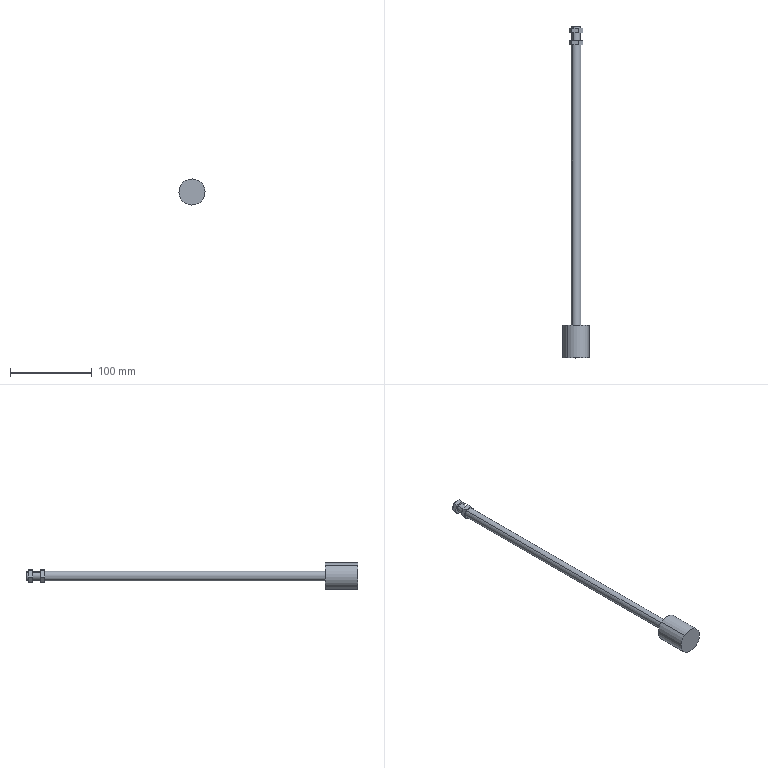Component | SolidWorks | A4-SDA 32X300-KC-L-1_A4-SDA 32X300-KC-L2-1 | 1 solid | 29 faces | box 32 x 407 x 32 mm | volume 73970 mm3 | plane 19 | cylinder 8 | cone 2 | commonest cylinder face diameters 10 x4 12 x2 32 x2
STEP:
#1=COLOUR_RGB('',0.7922,0.8196,0.9333);
#2=FILL_AREA_STYLE_COLOUR('',#1);
#3=FILL_AREA_STYLE('',(#2));
#4=SURFACE_STYLE_FILL_AREA(#3);
#5=SURFACE_SIDE_STYLE('',(#4));
#6=SURFACE_STYLE_USAGE(.BOTH.,#5);
#7=PRESENTATION_STYLE_ASSIGNMENT((#6));
#8=CARTESIAN_POINT('',(-0.1108,13.819,1.359));
#9=VERTEX_POINT('',#8);
#10=CARTESIAN_POINT('',(0.1108,13.819,1.082));
#11=VERTEX_POINT('',#10);
#12=CARTESIAN_POINT('',(-0.,13.819,1.22));
#13=DIRECTION('',(-0.,1.,0.));
#14=DIRECTION('',(-0.6255,0.,0.7802));
#15=AXIS2_PLACEMENT_3D('',#12,#13,#14);
#16=CIRCLE('',#15,0.1772);
#17=EDGE_CURVE('',#9,#11,#16,.T.);
#18=ORIENTED_EDGE('',*,*,#17,.F.);
#19=CARTESIAN_POINT('',(-0.1231,13.799,1.374));
#20=VERTEX_POINT('',#19);
#21=CARTESIAN_POINT('',(-0.1108,13.819,1.359));
#22=DIRECTION('',(-0.4423,-0.7071,0.5517));
#23=VECTOR('',#22,39.37);
#24=LINE('',#21,#23);
#25=EDGE_CURVE('',#9,#20,#24,.T.);
#26=ORIENTED_EDGE('',*,*,#25,.T.);
#27=CARTESIAN_POINT('',(0.1231,13.799,1.067));
#28=VERTEX_POINT('',#27);
#29=CARTESIAN_POINT('',(-0.,13.799,1.22));
#30=DIRECTION('',(0.,-1.,-0.));
#31=DIRECTION('',(-0.6255,0.,0.7802));
#32=AXIS2_PLACEMENT_3D('',#29,#30,#31);
#33=CIRCLE('',#32,0.1969);
#34=EDGE_CURVE('',#28,#20,#33,.T.);
#35=ORIENTED_EDGE('',*,*,#34,.F.);
#36=CARTESIAN_POINT('',(0.1108,13.819,1.082));
#37=DIRECTION('',(0.4423,-0.7071,-0.5517));
#38=VECTOR('',#37,39.37);
#39=LINE('',#36,#38);
#40=EDGE_CURVE('',#11,#28,#39,.T.);
#41=ORIENTED_EDGE('',*,*,#40,.F.);
#42=EDGE_LOOP('',(#18,#26,#35,#41));
#43=FACE_OUTER_BOUND('',#42,.T.);
#44=CARTESIAN_POINT('',(-0.,13.819,1.22));
#45=DIRECTION('',(0.,-1.,-0.));
#46=DIRECTION('',(0.6255,0.,-0.7802));
#47=AXIS2_PLACEMENT_3D('',#44,#45,#46);
#48=CONICAL_SURFACE('',#47,0.1772,0.7854);
#49=ADVANCED_FACE('',(#43),#48,.T.);
#50=CARTESIAN_POINT('',(-0.1478,12.913,1.405));
#51=VERTEX_POINT('',#50);
#52=CARTESIAN_POINT('',(0.1478,12.913,1.036));
#53=VERTEX_POINT('',#52);
#54=CARTESIAN_POINT('',(-0.,12.913,1.22));
#55=DIRECTION('',(-0.,1.,0.));
#56=DIRECTION('',(-0.6255,0.,0.7802));
#57=AXIS2_PLACEMENT_3D('',#54,#55,#56);
#58=CIRCLE('',#57,0.2362);
#59=EDGE_CURVE('',#51,#53,#58,.T.);
#60=ORIENTED_EDGE('',*,*,#59,.F.);
#61=CARTESIAN_POINT('',(-0.1478,-0.6299,1.405));
#62=VERTEX_POINT('',#61);
#63=CARTESIAN_POINT('',(-0.1478,12.913,1.405));
#64=DIRECTION('',(0.,-1.,-0.));
#65=VECTOR('',#64,39.37);
#66=LINE('',#63,#65);
#67=EDGE_CURVE('',#51,#62,#66,.T.);
#68=ORIENTED_EDGE('',*,*,#67,.T.);
#69=CARTESIAN_POINT('',(0.1478,-0.6299,1.036));
#70=VERTEX_POINT('',#69);
#71=CARTESIAN_POINT('',(0.,-0.6299,1.22));
#72=DIRECTION('',(-0.,1.,0.));
#73=DIRECTION('',(-0.6255,0.,0.7802));
#74=AXIS2_PLACEMENT_3D('',#71,#72,#73);
#75=CIRCLE('',#74,0.2362);
#76=EDGE_CURVE('',#62,#70,#75,.T.);
#77=ORIENTED_EDGE('',*,*,#76,.T.);
#78=CARTESIAN_POINT('',(0.1478,12.913,1.036));
#79=DIRECTION('',(0.,-1.,-0.));
#80=VECTOR('',#79,39.37);
#81=LINE('',#78,#80);
#82=EDGE_CURVE('',#53,#70,#81,.T.);
#83=ORIENTED_EDGE('',*,*,#82,.F.);
#84=EDGE_LOOP('',(#60,#68,#77,#83));
#85=FACE_OUTER_BOUND('',#84,.T.);
#86=CARTESIAN_POINT('',(-0.,12.913,1.22));
#87=DIRECTION('',(0.,-1.,-0.));
#88=DIRECTION('',(0.6255,0.,-0.7802));
#89=AXIS2_PLACEMENT_3D('',#86,#87,#88);
#90=CYLINDRICAL_SURFACE('',#89,0.2362);
#91=ADVANCED_FACE('',(#85),#90,.T.);
#92=CARTESIAN_POINT('',(-0.394,-2.205,1.712));
#93=VERTEX_POINT('',#92);
#94=CARTESIAN_POINT('',(0.394,-2.205,0.729));
#95=VERTEX_POINT('',#94);
#96=CARTESIAN_POINT('',(0.,-2.205,1.22));
#97=DIRECTION('',(-0.,1.,0.));
#98=DIRECTION('',(-0.6255,-0.,0.7802));
#99=AXIS2_PLACEMENT_3D('',#96,#97,#98);
#100=CIRCLE('',#99,0.6299);
#101=EDGE_CURVE('',#93,#95,#100,.T.);
#102=ORIENTED_EDGE('',*,*,#101,.T.);
#103=CARTESIAN_POINT('',(0.394,-0.6299,0.729));
#104=VERTEX_POINT('',#103);
#105=CARTESIAN_POINT('',(0.394,-2.205,0.729));
#106=DIRECTION('',(-0.,1.,0.));
#107=VECTOR('',#106,39.37);
#108=LINE('',#105,#107);
#109=EDGE_CURVE('',#95,#104,#108,.T.);
#110=ORIENTED_EDGE('',*,*,#109,.T.);
#111=CARTESIAN_POINT('',(-0.394,-0.6299,1.712));
#112=VERTEX_POINT('',#111);
#113=CARTESIAN_POINT('',(0.,-0.6299,1.22));
#114=DIRECTION('',(-0.,1.,0.));
#115=DIRECTION('',(-0.6255,-0.,0.7802));
#116=AXIS2_PLACEMENT_3D('',#113,#114,#115);
#117=CIRCLE('',#116,0.6299);
#118=EDGE_CURVE('',#112,#104,#117,.T.);
#119=ORIENTED_EDGE('',*,*,#118,.F.);
#120=CARTESIAN_POINT('',(-0.394,-2.205,1.712));
#121=DIRECTION('',(-0.,1.,0.));
#122=VECTOR('',#121,39.37);
#123=LINE('',#120,#122);
#124=EDGE_CURVE('',#93,#112,#123,.T.);
#125=ORIENTED_EDGE('',*,*,#124,.F.);
#126=EDGE_LOOP('',(#102,#110,#119,#125));
#127=FACE_OUTER_BOUND('',#126,.T.);
#128=CARTESIAN_POINT('',(0.,-2.205,1.22));
#129=DIRECTION('',(-0.,1.,0.));
#130=DIRECTION('',(-0.6255,-0.,0.7802));
#131=AXIS2_PLACEMENT_3D('',#128,#129,#130);
#132=CYLINDRICAL_SURFACE('',#131,0.6299);
#133=ADVANCED_FACE('',(#127),#132,.T.);
#134=ORIENTED_EDGE('',*,*,#34,.T.);
#135=CARTESIAN_POINT('',(-0.1231,13.701,1.374));
#136=VERTEX_POINT('',#135);
#137=CARTESIAN_POINT('',(-0.1231,13.819,1.374));
#138=DIRECTION('',(0.,-1.,-0.));
#139=VECTOR('',#138,39.37);
#140=LINE('',#137,#139);
#141=EDGE_CURVE('',#20,#136,#140,.T.);
#142=ORIENTED_EDGE('',*,*,#141,.T.);
#143=CARTESIAN_POINT('',(0.1231,13.701,1.067));
#144=VERTEX_POINT('',#143);
#145=CARTESIAN_POINT('',(-0.,13.701,1.22));
#146=DIRECTION('',(0.,-1.,-0.));
#147=DIRECTION('',(0.6255,0.,-0.7802));
#148=AXIS2_PLACEMENT_3D('',#145,#146,#147);
#149=CIRCLE('',#148,0.1969);
#150=EDGE_CURVE('',#144,#136,#149,.T.);
#151=ORIENTED_EDGE('',*,*,#150,.F.);
#152=CARTESIAN_POINT('',(0.1231,13.819,1.067));
#153=DIRECTION('',(0.,-1.,-0.));
#154=VECTOR('',#153,39.37);
#155=LINE('',#152,#154);
#156=EDGE_CURVE('',#28,#144,#155,.T.);
#157=ORIENTED_EDGE('',*,*,#156,.F.);
#158=EDGE_LOOP('',(#134,#142,#151,#157));
#159=FACE_OUTER_BOUND('',#158,.T.);
#160=CARTESIAN_POINT('',(-0.,13.819,1.22));
#161=DIRECTION('',(0.,-1.,-0.));
#162=DIRECTION('',(0.6255,0.,-0.7802));
#163=AXIS2_PLACEMENT_3D('',#160,#161,#162);
#164=CYLINDRICAL_SURFACE('',#163,0.1969);
#165=ADVANCED_FACE('',(#159),#164,.T.);
#166=CARTESIAN_POINT('',(0.1231,13.504,1.067));
#167=VERTEX_POINT('',#166);
#168=CARTESIAN_POINT('',(-0.1231,13.504,1.374));
#169=VERTEX_POINT('',#168);
#170=CARTESIAN_POINT('',(-0.,13.504,1.22));
#171=DIRECTION('',(0.,-1.,-0.));
#172=DIRECTION('',(0.6255,0.,-0.7802));
#173=AXIS2_PLACEMENT_3D('',#170,#171,#172);
#174=CIRCLE('',#173,0.1969);
#175=EDGE_CURVE('',#167,#169,#174,.T.);
#176=ORIENTED_EDGE('',*,*,#175,.T.);
#177=CARTESIAN_POINT('',(-0.1231,13.11,1.374));
#178=VERTEX_POINT('',#177);
#179=CARTESIAN_POINT('',(-0.1231,13.819,1.374));
#180=DIRECTION('',(0.,-1.,-0.));
#181=VECTOR('',#180,39.37);
#182=LINE('',#179,#181);
#183=EDGE_CURVE('',#169,#178,#182,.T.);
#184=ORIENTED_EDGE('',*,*,#183,.T.);
#185=CARTESIAN_POINT('',(0.1231,13.11,1.067));
#186=VERTEX_POINT('',#185);
#187=CARTESIAN_POINT('',(-0.,13.11,1.22));
#188=DIRECTION('',(0.,-1.,-0.));
#189=DIRECTION('',(0.6255,0.,-0.7802));
#190=AXIS2_PLACEMENT_3D('',#187,#188,#189);
#191=CIRCLE('',#190,0.1969);
#192=EDGE_CURVE('',#186,#178,#191,.T.);
#193=ORIENTED_EDGE('',*,*,#192,.F.);
#194=CARTESIAN_POINT('',(0.1231,13.819,1.067));
#195=DIRECTION('',(0.,-1.,-0.));
#196=VECTOR('',#195,39.37);
#197=LINE('',#194,#196);
#198=EDGE_CURVE('',#167,#186,#197,.T.);
#199=ORIENTED_EDGE('',*,*,#198,.F.);
#200=EDGE_LOOP('',(#176,#184,#193,#199));
#201=FACE_OUTER_BOUND('',#200,.T.);
#202=CARTESIAN_POINT('',(-0.,13.819,1.22));
#203=DIRECTION('',(0.,-1.,-0.));
#204=DIRECTION('',(0.6255,0.,-0.7802));
#205=AXIS2_PLACEMENT_3D('',#202,#203,#204);
#206=CYLINDRICAL_SURFACE('',#205,0.1969);
#207=ADVANCED_FACE('',(#201),#206,.T.);
#208=ORIENTED_EDGE('',*,*,#183,.F.);
#209=CARTESIAN_POINT('',(-0.,13.504,1.22));
#210=DIRECTION('',(0.,-1.,-0.));
#211=DIRECTION('',(0.6255,0.,-0.7802));
#212=AXIS2_PLACEMENT_3D('',#209,#210,#211);
#213=CIRCLE('',#212,0.1969);
#214=EDGE_CURVE('',#169,#167,#213,.T.);
#215=ORIENTED_EDGE('',*,*,#214,.T.);
#216=ORIENTED_EDGE('',*,*,#198,.T.);
#217=CARTESIAN_POINT('',(-0.,13.11,1.22));
#218=DIRECTION('',(0.,-1.,-0.));
#219=DIRECTION('',(0.6255,0.,-0.7802));
#220=AXIS2_PLACEMENT_3D('',#217,#218,#219);
#221=CIRCLE('',#220,0.1969);
#222=EDGE_CURVE('',#178,#186,#221,.T.);
#223=ORIENTED_EDGE('',*,*,#222,.F.);
#224=EDGE_LOOP('',(#208,#215,#216,#223));
#225=FACE_OUTER_BOUND('',#224,.T.);
#226=CARTESIAN_POINT('',(-0.,13.819,1.22));
#227=DIRECTION('',(0.,-1.,-0.));
#228=DIRECTION('',(0.6255,0.,-0.7802));
#229=AXIS2_PLACEMENT_3D('',#226,#227,#228);
#230=CYLINDRICAL_SURFACE('',#229,0.1969);
#231=ADVANCED_FACE('',(#225),#230,.T.);
#232=CARTESIAN_POINT('',(0.3308,13.504,1.271));
#233=VERTEX_POINT('',#232);
#234=CARTESIAN_POINT('',(0.2093,13.504,0.9594));
#235=VERTEX_POINT('',#234);
#236=CARTESIAN_POINT('',(0.2093,13.504,0.9594));
#237=DIRECTION('',(-0.363,0.,-0.9318));
#238=VECTOR('',#237,39.37);
#239=LINE('',#236,#238);
#240=EDGE_CURVE('',#233,#235,#239,.T.);
#241=ORIENTED_EDGE('',*,*,#240,.F.);
#242=CARTESIAN_POINT('',(0.1215,13.504,1.532));
#243=VERTEX_POINT('',#242);
#244=CARTESIAN_POINT('',(0.3308,13.504,1.271));
#245=DIRECTION('',(0.6255,0.,-0.7802));
#246=VECTOR('',#245,39.37);
#247=LINE('',#244,#246);
#248=EDGE_CURVE('',#243,#233,#247,.T.);
#249=ORIENTED_EDGE('',*,*,#248,.F.);
#250=CARTESIAN_POINT('',(-0.2093,13.504,1.482));
#251=VERTEX_POINT('',#250);
#252=CARTESIAN_POINT('',(0.1215,13.504,1.532));
#253=DIRECTION('',(0.9884,0.,0.1516));
#254=VECTOR('',#253,39.37);
#255=LINE('',#252,#254);
#256=EDGE_CURVE('',#251,#243,#255,.T.);
#257=ORIENTED_EDGE('',*,*,#256,.F.);
#258=CARTESIAN_POINT('',(-0.3308,13.504,1.17));
#259=VERTEX_POINT('',#258);
#260=CARTESIAN_POINT('',(-0.2093,13.504,1.482));
#261=DIRECTION('',(0.363,-0.,0.9318));
#262=VECTOR('',#261,39.37);
#263=LINE('',#260,#262);
#264=EDGE_CURVE('',#259,#251,#263,.T.);
#265=ORIENTED_EDGE('',*,*,#264,.F.);
#266=CARTESIAN_POINT('',(-0.1215,13.504,0.9086));
#267=VERTEX_POINT('',#266);
#268=CARTESIAN_POINT('',(-0.3308,13.504,1.17));
#269=DIRECTION('',(-0.6255,-0.,0.7802));
#270=VECTOR('',#269,39.37);
#271=LINE('',#268,#270);
#272=EDGE_CURVE('',#267,#259,#271,.T.);
#273=ORIENTED_EDGE('',*,*,#272,.F.);
#274=CARTESIAN_POINT('',(-0.1215,13.504,0.9086));
#275=DIRECTION('',(-0.9884,-0.,-0.1516));
#276=VECTOR('',#275,39.37);
#277=LINE('',#274,#276);
#278=EDGE_CURVE('',#235,#267,#277,.T.);
#279=ORIENTED_EDGE('',*,*,#278,.F.);
#280=EDGE_LOOP('',(#241,#249,#257,#265,#273,#279));
#281=FACE_OUTER_BOUND('',#280,.T.);
#282=ORIENTED_EDGE('',*,*,#175,.F.);
#283=ORIENTED_EDGE('',*,*,#214,.F.);
#284=EDGE_LOOP('',(#282,#283));
#285=FACE_BOUND('',#284,.T.);
#286=CARTESIAN_POINT('',(-0.,13.504,1.22));
#287=DIRECTION('',(0.,-1.,-0.));
#288=DIRECTION('',(0.6255,0.,-0.7802));
#289=AXIS2_PLACEMENT_3D('',#286,#287,#288);
#290=PLANE('',#289);
#291=ADVANCED_FACE('',(#281,#285),#290,.T.);
#292=CARTESIAN_POINT('',(0.3308,13.701,1.271));
#293=VERTEX_POINT('',#292);
#294=CARTESIAN_POINT('',(0.2093,13.701,0.9594));
#295=VERTEX_POINT('',#294);
#296=CARTESIAN_POINT('',(0.2093,13.701,0.9594));
#297=DIRECTION('',(-0.363,0.,-0.9318));
#298=VECTOR('',#297,39.37);
#299=LINE('',#296,#298);
#300=EDGE_CURVE('',#293,#295,#299,.T.);
#301=ORIENTED_EDGE('',*,*,#300,.T.);
#302=CARTESIAN_POINT('',(-0.1215,13.701,0.9086));
#303=VERTEX_POINT('',#302);
#304=CARTESIAN_POINT('',(-0.1215,13.701,0.9086));
#305=DIRECTION('',(-0.9884,-0.,-0.1516));
#306=VECTOR('',#305,39.37);
#307=LINE('',#304,#306);
#308=EDGE_CURVE('',#295,#303,#307,.T.);
#309=ORIENTED_EDGE('',*,*,#308,.T.);
#310=CARTESIAN_POINT('',(-0.3308,13.701,1.17));
#311=VERTEX_POINT('',#310);
#312=CARTESIAN_POINT('',(-0.3308,13.701,1.17));
#313=DIRECTION('',(-0.6255,-0.,0.7802));
#314=VECTOR('',#313,39.37);
#315=LINE('',#312,#314);
#316=EDGE_CURVE('',#303,#311,#315,.T.);
#317=ORIENTED_EDGE('',*,*,#316,.T.);
#318=CARTESIAN_POINT('',(-0.2093,13.701,1.482));
#319=VERTEX_POINT('',#318);
#320=CARTESIAN_POINT('',(-0.2093,13.701,1.482));
#321=DIRECTION('',(0.363,-0.,0.9318));
#322=VECTOR('',#321,39.37);
#323=LINE('',#320,#322);
#324=EDGE_CURVE('',#311,#319,#323,.T.);
#325=ORIENTED_EDGE('',*,*,#324,.T.);
#326=CARTESIAN_POINT('',(0.1215,13.701,1.532));
#327=VERTEX_POINT('',#326);
#328=CARTESIAN_POINT('',(0.1215,13.701,1.532));
#329=DIRECTION('',(0.9884,0.,0.1516));
#330=VECTOR('',#329,39.37);
#331=LINE('',#328,#330);
#332=EDGE_CURVE('',#319,#327,#331,.T.);
#333=ORIENTED_EDGE('',*,*,#332,.T.);
#334=CARTESIAN_POINT('',(0.3308,13.701,1.271));
#335=DIRECTION('',(0.6255,0.,-0.7802));
#336=VECTOR('',#335,39.37);
#337=LINE('',#334,#336);
#338=EDGE_CURVE('',#327,#293,#337,.T.);
#339=ORIENTED_EDGE('',*,*,#338,.T.);
#340=EDGE_LOOP('',(#301,#309,#317,#325,#333,#339));
#341=FACE_OUTER_BOUND('',#340,.T.);
#342=ORIENTED_EDGE('',*,*,#150,.T.);
#343=CARTESIAN_POINT('',(-0.,13.701,1.22));
#344=DIRECTION('',(0.,-1.,-0.));
#345=DIRECTION('',(0.6255,0.,-0.7802));
#346=AXIS2_PLACEMENT_3D('',#343,#344,#345);
#347=CIRCLE('',#346,0.1969);
#348=EDGE_CURVE('',#136,#144,#347,.T.);
#349=ORIENTED_EDGE('',*,*,#348,.T.);
#350=EDGE_LOOP('',(#342,#349));
#351=FACE_BOUND('',#350,.T.);
#352=CARTESIAN_POINT('',(-0.,13.701,1.22));
#353=DIRECTION('',(0.,-1.,-0.));
#354=DIRECTION('',(0.6255,0.,-0.7802));
#355=AXIS2_PLACEMENT_3D('',#352,#353,#354);
#356=PLANE('',#355);
#357=ADVANCED_FACE('',(#341,#351),#356,.F.);
#358=ORIENTED_EDGE('',*,*,#300,.F.);
#359=CARTESIAN_POINT('',(0.3308,13.504,1.271));
#360=DIRECTION('',(-0.,1.,0.));
#361=VECTOR('',#360,39.37);
#362=LINE('',#359,#361);
#363=EDGE_CURVE('',#233,#293,#362,.T.);
#364=ORIENTED_EDGE('',*,*,#363,.F.);
#365=ORIENTED_EDGE('',*,*,#240,.T.);
#366=CARTESIAN_POINT('',(0.2093,13.504,0.9594));
#367=DIRECTION('',(-0.,1.,0.));
#368=VECTOR('',#367,39.37);
#369=LINE('',#366,#368);
#370=EDGE_CURVE('',#235,#295,#369,.T.);
#371=ORIENTED_EDGE('',*,*,#370,.T.);
#372=EDGE_LOOP('',(#358,#364,#365,#371));
#373=FACE_OUTER_BOUND('',#372,.T.);
#374=CARTESIAN_POINT('',(0.2093,13.504,0.9594));
#375=DIRECTION('',(0.9318,0.,-0.363));
#376=DIRECTION('',(-0.363,0.,-0.9318));
#377=AXIS2_PLACEMENT_3D('',#374,#375,#376);
#378=PLANE('',#377);
#379=ADVANCED_FACE('',(#373),#378,.T.);
#380=ORIENTED_EDGE('',*,*,#338,.F.);
#381=CARTESIAN_POINT('',(0.1215,13.504,1.532));
#382=DIRECTION('',(-0.,1.,0.));
#383=VECTOR('',#382,39.37);
#384=LINE('',#381,#383);
#385=EDGE_CURVE('',#243,#327,#384,.T.);
#386=ORIENTED_EDGE('',*,*,#385,.F.);
#387=ORIENTED_EDGE('',*,*,#248,.T.);
#388=ORIENTED_EDGE('',*,*,#363,.T.);
#389=EDGE_LOOP('',(#380,#386,#387,#388));
#390=FACE_OUTER_BOUND('',#389,.T.);
#391=CARTESIAN_POINT('',(0.3308,13.504,1.271));
#392=DIRECTION('',(0.7802,0.,0.6255));
#393=DIRECTION('',(-0.,1.,0.));
#394=AXIS2_PLACEMENT_3D('',#391,#392,#393);
#395=PLANE('',#394);
#396=ADVANCED_FACE('',(#390),#395,.T.);
#397=ORIENTED_EDGE('',*,*,#332,.F.);
#398=CARTESIAN_POINT('',(-0.2093,13.504,1.482));
#399=DIRECTION('',(-0.,1.,0.));
#400=VECTOR('',#399,39.37);
#401=LINE('',#398,#400);
#402=EDGE_CURVE('',#251,#319,#401,.T.);
#403=ORIENTED_EDGE('',*,*,#402,.F.);
#404=ORIENTED_EDGE('',*,*,#256,.T.);
#405=ORIENTED_EDGE('',*,*,#385,.T.);
#406=EDGE_LOOP('',(#397,#403,#404,#405));
#407=FACE_OUTER_BOUND('',#406,.T.);
#408=CARTESIAN_POINT('',(0.1215,13.504,1.532));
#409=DIRECTION('',(-0.1516,-0.,0.9884));
#410=DIRECTION('',(0.9884,0.,0.1516));
#411=AXIS2_PLACEMENT_3D('',#408,#409,#410);
#412=PLANE('',#411);
#413=ADVANCED_FACE('',(#407),#412,.T.);
#414=ORIENTED_EDGE('',*,*,#324,.F.);
#415=CARTESIAN_POINT('',(-0.3308,13.504,1.17));
#416=DIRECTION('',(-0.,1.,0.));
#417=VECTOR('',#416,39.37);
#418=LINE('',#415,#417);
#419=EDGE_CURVE('',#259,#311,#418,.T.);
#420=ORIENTED_EDGE('',*,*,#419,.F.);
#421=ORIENTED_EDGE('',*,*,#264,.T.);
#422=ORIENTED_EDGE('',*,*,#402,.T.);
#423=EDGE_LOOP('',(#414,#420,#421,#422));
#424=FACE_OUTER_BOUND('',#423,.T.);
#425=CARTESIAN_POINT('',(-0.2093,13.504,1.482));
#426=DIRECTION('',(-0.9318,-0.,0.363));
#427=DIRECTION('',(0.363,-0.,0.9318));
#428=AXIS2_PLACEMENT_3D('',#425,#426,#427);
#429=PLANE('',#428);
#430=ADVANCED_FACE('',(#424),#429,.T.);
#431=ORIENTED_EDGE('',*,*,#316,.F.);
#432=CARTESIAN_POINT('',(-0.1215,13.504,0.9086));
#433=DIRECTION('',(-0.,1.,0.));
#434=VECTOR('',#433,39.37);
#435=LINE('',#432,#434);
#436=EDGE_CURVE('',#267,#303,#435,.T.);
#437=ORIENTED_EDGE('',*,*,#436,.F.);
#438=ORIENTED_EDGE('',*,*,#272,.T.);
#439=ORIENTED_EDGE('',*,*,#419,.T.);
#440=EDGE_LOOP('',(#431,#437,#438,#439));
#441=FACE_OUTER_BOUND('',#440,.T.);
#442=CARTESIAN_POINT('',(-0.3308,13.504,1.17));
#443=DIRECTION('',(-0.7802,-0.,-0.6255));
#444=DIRECTION('',(0.,-1.,-0.));
#445=AXIS2_PLACEMENT_3D('',#442,#443,#444);
#446=PLANE('',#445);
#447=ADVANCED_FACE('',(#441),#446,.T.);
#448=ORIENTED_EDGE('',*,*,#308,.F.);
#449=ORIENTED_EDGE('',*,*,#370,.F.);
#450=ORIENTED_EDGE('',*,*,#278,.T.);
#451=ORIENTED_EDGE('',*,*,#436,.T.);
#452=EDGE_LOOP('',(#448,#449,#450,#451));
#453=FACE_OUTER_BOUND('',#452,.T.);
#454=CARTESIAN_POINT('',(-0.1215,13.504,0.9086));
#455=DIRECTION('',(0.1516,0.,-0.9884));
#456=DIRECTION('',(-0.9884,-0.,-0.1516));
#457=AXIS2_PLACEMENT_3D('',#454,#455,#456);
#458=PLANE('',#457);
#459=ADVANCED_FACE('',(#453),#458,.T.);
#460=CARTESIAN_POINT('',(-0.,13.819,1.22));
#461=DIRECTION('',(-0.,1.,0.));
#462=DIRECTION('',(-0.6255,0.,0.7802));
#463=AXIS2_PLACEMENT_3D('',#460,#461,#462);
#464=CIRCLE('',#463,0.1772);
#465=EDGE_CURVE('',#11,#9,#464,.T.);
#466=ORIENTED_EDGE('',*,*,#465,.T.);
#467=ORIENTED_EDGE('',*,*,#17,.T.);
#468=EDGE_LOOP('',(#466,#467));
#469=FACE_OUTER_BOUND('',#468,.T.);
#470=CARTESIAN_POINT('',(-0.,13.819,1.22));
#471=DIRECTION('',(-0.,1.,0.));
#472=DIRECTION('',(-0.6255,-0.,0.7802));
#473=AXIS2_PLACEMENT_3D('',#470,#471,#472);
#474=PLANE('',#473);
#475=ADVANCED_FACE('',(#469),#474,.T.);
#476=ORIENTED_EDGE('',*,*,#141,.F.);
#477=CARTESIAN_POINT('',(-0.,13.799,1.22));
#478=DIRECTION('',(0.,-1.,-0.));
#479=DIRECTION('',(-0.6255,0.,0.7802));
#480=AXIS2_PLACEMENT_3D('',#477,#478,#479);
#481=CIRCLE('',#480,0.1969);
#482=EDGE_CURVE('',#20,#28,#481,.T.);
#483=ORIENTED_EDGE('',*,*,#482,.T.);
#484=ORIENTED_EDGE('',*,*,#156,.T.);
#485=ORIENTED_EDGE('',*,*,#348,.F.);
#486=EDGE_LOOP('',(#476,#483,#484,#485));
#487=FACE_OUTER_BOUND('',#486,.T.);
#488=CARTESIAN_POINT('',(-0.,13.819,1.22));
#489=DIRECTION('',(0.,-1.,-0.));
#490=DIRECTION('',(0.6255,0.,-0.7802));
#491=AXIS2_PLACEMENT_3D('',#488,#489,#490);
#492=CYLINDRICAL_SURFACE('',#491,0.1969);
#493=ADVANCED_FACE('',(#487),#492,.T.);
#494=CARTESIAN_POINT('',(0.3308,12.913,1.271));
#495=VERTEX_POINT('',#494);
#496=CARTESIAN_POINT('',(0.2093,12.913,0.9594));
#497=VERTEX_POINT('',#496);
#498=CARTESIAN_POINT('',(0.2093,12.913,0.9594));
#499=DIRECTION('',(-0.363,0.,-0.9318));
#500=VECTOR('',#499,39.37);
#501=LINE('',#498,#500);
#502=EDGE_CURVE('',#495,#497,#501,.T.);
#503=ORIENTED_EDGE('',*,*,#502,.F.);
#504=CARTESIAN_POINT('',(0.1215,12.913,1.532));
#505=VERTEX_POINT('',#504);
#506=CARTESIAN_POINT('',(0.3308,12.913,1.271));
#507=DIRECTION('',(0.6255,0.,-0.7802));
#508=VECTOR('',#507,39.37);
#509=LINE('',#506,#508);
#510=EDGE_CURVE('',#505,#495,#509,.T.);
#511=ORIENTED_EDGE('',*,*,#510,.F.);
#512=CARTESIAN_POINT('',(-0.2093,12.913,1.482));
#513=VERTEX_POINT('',#512);
#514=CARTESIAN_POINT('',(0.1215,12.913,1.532));
#515=DIRECTION('',(0.9884,0.,0.1516));
#516=VECTOR('',#515,39.37);
#517=LINE('',#514,#516);
#518=EDGE_CURVE('',#513,#505,#517,.T.);
#519=ORIENTED_EDGE('',*,*,#518,.F.);
#520=CARTESIAN_POINT('',(-0.3308,12.913,1.17));
#521=VERTEX_POINT('',#520);
#522=CARTESIAN_POINT('',(-0.2093,12.913,1.482));
#523=DIRECTION('',(0.363,-0.,0.9318));
#524=VECTOR('',#523,39.37);
#525=LINE('',#522,#524);
#526=EDGE_CURVE('',#521,#513,#525,.T.);
#527=ORIENTED_EDGE('',*,*,#526,.F.);
#528=CARTESIAN_POINT('',(-0.1215,12.913,0.9086));
#529=VERTEX_POINT('',#528);
#530=CARTESIAN_POINT('',(-0.3308,12.913,1.17));
#531=DIRECTION('',(-0.6255,-0.,0.7802));
#532=VECTOR('',#531,39.37);
#533=LINE('',#530,#532);
#534=EDGE_CURVE('',#529,#521,#533,.T.);
#535=ORIENTED_EDGE('',*,*,#534,.F.);
#536=CARTESIAN_POINT('',(-0.1215,12.913,0.9086));
#537=DIRECTION('',(-0.9884,-0.,-0.1516));
#538=VECTOR('',#537,39.37);
#539=LINE('',#536,#538);
#540=EDGE_CURVE('',#497,#529,#539,.T.);
#541=ORIENTED_EDGE('',*,*,#540,.F.);
#542=EDGE_LOOP('',(#503,#511,#519,#527,#535,#541));
#543=FACE_OUTER_BOUND('',#542,.T.);
#544=CARTESIAN_POINT('',(-0.,12.913,1.22));
#545=DIRECTION('',(-0.,1.,0.));
#546=DIRECTION('',(-0.6255,0.,0.7802));
#547=AXIS2_PLACEMENT_3D('',#544,#545,#546);
#548=CIRCLE('',#547,0.2362);
#549=EDGE_CURVE('',#53,#51,#548,.T.);
#550=ORIENTED_EDGE('',*,*,#549,.T.);
#551=ORIENTED_EDGE('',*,*,#59,.T.);
#552=EDGE_LOOP('',(#550,#551));
#553=FACE_BOUND('',#552,.T.);
#554=CARTESIAN_POINT('',(-0.,12.913,1.22));
#555=DIRECTION('',(0.,-1.,-0.));
#556=DIRECTION('',(0.6255,0.,-0.7802));
#557=AXIS2_PLACEMENT_3D('',#554,#555,#556);
#558=PLANE('',#557);
#559=ADVANCED_FACE('',(#543,#553),#558,.T.);
#560=CARTESIAN_POINT('',(0.3308,13.11,1.271));
#561=VERTEX_POINT('',#560);
#562=CARTESIAN_POINT('',(0.2093,13.11,0.9594));
#563=VERTEX_POINT('',#562);
#564=CARTESIAN_POINT('',(0.2093,13.11,0.9594));
#565=DIRECTION('',(-0.363,0.,-0.9318));
#566=VECTOR('',#565,39.37);
#567=LINE('',#564,#566);
#568=EDGE_CURVE('',#561,#563,#567,.T.);
#569=ORIENTED_EDGE('',*,*,#568,.T.);
#570=CARTESIAN_POINT('',(-0.1215,13.11,0.9086));
#571=VERTEX_POINT('',#570);
#572=CARTESIAN_POINT('',(-0.1215,13.11,0.9086));
#573=DIRECTION('',(-0.9884,-0.,-0.1516));
#574=VECTOR('',#573,39.37);
#575=LINE('',#572,#574);
#576=EDGE_CURVE('',#563,#571,#575,.T.);
#577=ORIENTED_EDGE('',*,*,#576,.T.);
#578=CARTESIAN_POINT('',(-0.3308,13.11,1.17));
#579=VERTEX_POINT('',#578);
#580=CARTESIAN_POINT('',(-0.3308,13.11,1.17));
#581=DIRECTION('',(-0.6255,-0.,0.7802));
#582=VECTOR('',#581,39.37);
#583=LINE('',#580,#582);
#584=EDGE_CURVE('',#571,#579,#583,.T.);
#585=ORIENTED_EDGE('',*,*,#584,.T.);
#586=CARTESIAN_POINT('',(-0.2093,13.11,1.482));
#587=VERTEX_POINT('',#586);
#588=CARTESIAN_POINT('',(-0.2093,13.11,1.482));
#589=DIRECTION('',(0.363,-0.,0.9318));
#590=VECTOR('',#589,39.37);
#591=LINE('',#588,#590);
#592=EDGE_CURVE('',#579,#587,#591,.T.);
#593=ORIENTED_EDGE('',*,*,#592,.T.);
#594=CARTESIAN_POINT('',(0.1215,13.11,1.532));
#595=VERTEX_POINT('',#594);
#596=CARTESIAN_POINT('',(0.1215,13.11,1.532));
#597=DIRECTION('',(0.9884,0.,0.1516));
#598=VECTOR('',#597,39.37);
#599=LINE('',#596,#598);
#600=EDGE_CURVE('',#587,#595,#599,.T.);
#601=ORIENTED_EDGE('',*,*,#600,.T.);
#602=CARTESIAN_POINT('',(0.3308,13.11,1.271));
#603=DIRECTION('',(0.6255,0.,-0.7802));
#604=VECTOR('',#603,39.37);
#605=LINE('',#602,#604);
#606=EDGE_CURVE('',#595,#561,#605,.T.);
#607=ORIENTED_EDGE('',*,*,#606,.T.);
#608=EDGE_LOOP('',(#569,#577,#585,#593,#601,#607));
#609=FACE_OUTER_BOUND('',#608,.T.);
#610=ORIENTED_EDGE('',*,*,#192,.T.);
#611=ORIENTED_EDGE('',*,*,#222,.T.);
#612=EDGE_LOOP('',(#610,#611));
#613=FACE_BOUND('',#612,.T.);
#614=CARTESIAN_POINT('',(-0.,13.11,1.22));
#615=DIRECTION('',(0.,-1.,-0.));
#616=DIRECTION('',(0.6255,0.,-0.7802));
#617=AXIS2_PLACEMENT_3D('',#614,#615,#616);
#618=PLANE('',#617);
#619=ADVANCED_FACE('',(#609,#613),#618,.F.);
#620=ORIENTED_EDGE('',*,*,#568,.F.);
#621=CARTESIAN_POINT('',(0.3308,12.913,1.271));
#622=DIRECTION('',(-0.,1.,0.));
#623=VECTOR('',#622,39.37);
#624=LINE('',#621,#623);
#625=EDGE_CURVE('',#495,#561,#624,.T.);
#626=ORIENTED_EDGE('',*,*,#625,.F.);
#627=ORIENTED_EDGE('',*,*,#502,.T.);
#628=CARTESIAN_POINT('',(0.2093,12.913,0.9594));
#629=DIRECTION('',(-0.,1.,0.));
#630=VECTOR('',#629,39.37);
#631=LINE('',#628,#630);
#632=EDGE_CURVE('',#497,#563,#631,.T.);
#633=ORIENTED_EDGE('',*,*,#632,.T.);
#634=EDGE_LOOP('',(#620,#626,#627,#633));
#635=FACE_OUTER_BOUND('',#634,.T.);
#636=CARTESIAN_POINT('',(0.2093,12.913,0.9594));
#637=DIRECTION('',(0.9318,0.,-0.363));
#638=DIRECTION('',(-0.363,0.,-0.9318));
#639=AXIS2_PLACEMENT_3D('',#636,#637,#638);
#640=PLANE('',#639);
#641=ADVANCED_FACE('',(#635),#640,.T.);
#642=ORIENTED_EDGE('',*,*,#606,.F.);
#643=CARTESIAN_POINT('',(0.1215,12.913,1.532));
#644=DIRECTION('',(-0.,1.,0.));
#645=VECTOR('',#644,39.37);
#646=LINE('',#643,#645);
#647=EDGE_CURVE('',#505,#595,#646,.T.);
#648=ORIENTED_EDGE('',*,*,#647,.F.);
#649=ORIENTED_EDGE('',*,*,#510,.T.);
#650=ORIENTED_EDGE('',*,*,#625,.T.);
#651=EDGE_LOOP('',(#642,#648,#649,#650));
#652=FACE_OUTER_BOUND('',#651,.T.);
#653=CARTESIAN_POINT('',(0.3308,12.913,1.271));
#654=DIRECTION('',(0.7802,0.,0.6255));
#655=DIRECTION('',(-0.,1.,0.));
#656=AXIS2_PLACEMENT_3D('',#653,#654,#655);
#657=PLANE('',#656);
#658=ADVANCED_FACE('',(#652),#657,.T.);
#659=ORIENTED_EDGE('',*,*,#600,.F.);
#660=CARTESIAN_POINT('',(-0.2093,12.913,1.482));
#661=DIRECTION('',(-0.,1.,0.));
#662=VECTOR('',#661,39.37);
#663=LINE('',#660,#662);
#664=EDGE_CURVE('',#513,#587,#663,.T.);
#665=ORIENTED_EDGE('',*,*,#664,.F.);
#666=ORIENTED_EDGE('',*,*,#518,.T.);
#667=ORIENTED_EDGE('',*,*,#647,.T.);
#668=EDGE_LOOP('',(#659,#665,#666,#667));
#669=FACE_OUTER_BOUND('',#668,.T.);
#670=CARTESIAN_POINT('',(0.1215,12.913,1.532));
#671=DIRECTION('',(-0.1516,-0.,0.9884));
#672=DIRECTION('',(0.9884,0.,0.1516));
#673=AXIS2_PLACEMENT_3D('',#670,#671,#672);
#674=PLANE('',#673);
#675=ADVANCED_FACE('',(#669),#674,.T.);
#676=ORIENTED_EDGE('',*,*,#592,.F.);
#677=CARTESIAN_POINT('',(-0.3308,12.913,1.17));
#678=DIRECTION('',(-0.,1.,0.));
#679=VECTOR('',#678,39.37);
#680=LINE('',#677,#679);
#681=EDGE_CURVE('',#521,#579,#680,.T.);
#682=ORIENTED_EDGE('',*,*,#681,.F.);
#683=ORIENTED_EDGE('',*,*,#526,.T.);
#684=ORIENTED_EDGE('',*,*,#664,.T.);
#685=EDGE_LOOP('',(#676,#682,#683,#684));
#686=FACE_OUTER_BOUND('',#685,.T.);
#687=CARTESIAN_POINT('',(-0.2093,12.913,1.482));
#688=DIRECTION('',(-0.9318,-0.,0.363));
#689=DIRECTION('',(0.363,-0.,0.9318));
#690=AXIS2_PLACEMENT_3D('',#687,#688,#689);
#691=PLANE('',#690);
#692=ADVANCED_FACE('',(#686),#691,.T.);
#693=ORIENTED_EDGE('',*,*,#584,.F.);
#694=CARTESIAN_POINT('',(-0.1215,12.913,0.9086));
#695=DIRECTION('',(-0.,1.,0.));
#696=VECTOR('',#695,39.37);
#697=LINE('',#694,#696);
#698=EDGE_CURVE('',#529,#571,#697,.T.);
#699=ORIENTED_EDGE('',*,*,#698,.F.);
#700=ORIENTED_EDGE('',*,*,#534,.T.);
#701=ORIENTED_EDGE('',*,*,#681,.T.);
#702=EDGE_LOOP('',(#693,#699,#700,#701));
#703=FACE_OUTER_BOUND('',#702,.T.);
#704=CARTESIAN_POINT('',(-0.3308,12.913,1.17));
#705=DIRECTION('',(-0.7802,-0.,-0.6255));
#706=DIRECTION('',(0.,-1.,-0.));
#707=AXIS2_PLACEMENT_3D('',#704,#705,#706);
#708=PLANE('',#707);
#709=ADVANCED_FACE('',(#703),#708,.T.);
#710=ORIENTED_EDGE('',*,*,#576,.F.);
#711=ORIENTED_EDGE('',*,*,#632,.F.);
#712=ORIENTED_EDGE('',*,*,#540,.T.);
#713=ORIENTED_EDGE('',*,*,#698,.T.);
#714=EDGE_LOOP('',(#710,#711,#712,#713));
#715=FACE_OUTER_BOUND('',#714,.T.);
#716=CARTESIAN_POINT('',(-0.1215,12.913,0.9086));
#717=DIRECTION('',(0.1516,0.,-0.9884));
#718=DIRECTION('',(-0.9884,-0.,-0.1516));
#719=AXIS2_PLACEMENT_3D('',#716,#717,#718);
#720=PLANE('',#719);
#721=ADVANCED_FACE('',(#715),#720,.T.);
#722=ORIENTED_EDGE('',*,*,#101,.F.);
#723=CARTESIAN_POINT('',(0.,-2.205,1.22));
#724=DIRECTION('',(-0.,1.,0.));
#725=DIRECTION('',(-0.6255,-0.,0.7802));
#726=AXIS2_PLACEMENT_3D('',#723,#724,#725);
#727=CIRCLE('',#726,0.6299);
#728=EDGE_CURVE('',#95,#93,#727,.T.);
#729=ORIENTED_EDGE('',*,*,#728,.F.);
#730=EDGE_LOOP('',(#722,#729));
#731=FACE_OUTER_BOUND('',#730,.T.);
#732=CARTESIAN_POINT('',(0.,-2.205,1.22));
#733=DIRECTION('',(-0.,1.,0.));
#734=DIRECTION('',(-0.6255,-0.,0.7802));
#735=AXIS2_PLACEMENT_3D('',#732,#733,#734);
#736=PLANE('',#735);
#737=ADVANCED_FACE('',(#731),#736,.F.);
#738=ORIENTED_EDGE('',*,*,#109,.F.);
#739=ORIENTED_EDGE('',*,*,#728,.T.);
#740=ORIENTED_EDGE('',*,*,#124,.T.);
#741=CARTESIAN_POINT('',(0.,-0.6299,1.22));
#742=DIRECTION('',(-0.,1.,0.));
#743=DIRECTION('',(-0.6255,-0.,0.7802));
#744=AXIS2_PLACEMENT_3D('',#741,#742,#743);
#745=CIRCLE('',#744,0.6299);
#746=EDGE_CURVE('',#104,#112,#745,.T.);
#747=ORIENTED_EDGE('',*,*,#746,.F.);
#748=EDGE_LOOP('',(#738,#739,#740,#747));
#749=FACE_OUTER_BOUND('',#748,.T.);
#750=CARTESIAN_POINT('',(0.,-2.205,1.22));
#751=DIRECTION('',(-0.,1.,0.));
#752=DIRECTION('',(-0.6255,-0.,0.7802));
#753=AXIS2_PLACEMENT_3D('',#750,#751,#752);
#754=CYLINDRICAL_SURFACE('',#753,0.6299);
#755=ADVANCED_FACE('',(#749),#754,.T.);
#756=ORIENTED_EDGE('',*,*,#118,.T.);
#757=ORIENTED_EDGE('',*,*,#746,.T.);
#758=EDGE_LOOP('',(#756,#757));
#759=FACE_OUTER_BOUND('',#758,.T.);
#760=CARTESIAN_POINT('',(0.,-0.6299,1.22));
#761=DIRECTION('',(-0.,1.,0.));
#762=DIRECTION('',(-0.6255,0.,0.7802));
#763=AXIS2_PLACEMENT_3D('',#760,#761,#762);
#764=CIRCLE('',#763,0.2362);
#765=EDGE_CURVE('',#70,#62,#764,.T.);
#766=ORIENTED_EDGE('',*,*,#765,.F.);
#767=ORIENTED_EDGE('',*,*,#76,.F.);
#768=EDGE_LOOP('',(#766,#767));
#769=FACE_BOUND('',#768,.T.);
#770=CARTESIAN_POINT('',(0.,-0.6299,1.22));
#771=DIRECTION('',(-0.,1.,0.));
#772=DIRECTION('',(-0.6255,-0.,0.7802));
#773=AXIS2_PLACEMENT_3D('',#770,#771,#772);
#774=PLANE('',#773);
#775=ADVANCED_FACE('',(#759,#769),#774,.T.);
#776=ORIENTED_EDGE('',*,*,#67,.F.);
#777=ORIENTED_EDGE('',*,*,#549,.F.);
#778=ORIENTED_EDGE('',*,*,#82,.T.);
#779=ORIENTED_EDGE('',*,*,#765,.T.);
#780=EDGE_LOOP('',(#776,#777,#778,#779));
#781=FACE_OUTER_BOUND('',#780,.T.);
#782=CARTESIAN_POINT('',(-0.,12.913,1.22));
#783=DIRECTION('',(0.,-1.,-0.));
#784=DIRECTION('',(0.6255,0.,-0.7802));
#785=AXIS2_PLACEMENT_3D('',#782,#783,#784);
#786=CYLINDRICAL_SURFACE('',#785,0.2362);
#787=ADVANCED_FACE('',(#781),#786,.T.);
#788=ORIENTED_EDGE('',*,*,#25,.F.);
#789=ORIENTED_EDGE('',*,*,#465,.F.);
#790=ORIENTED_EDGE('',*,*,#40,.T.);
#791=ORIENTED_EDGE('',*,*,#482,.F.);
#792=EDGE_LOOP('',(#788,#789,#790,#791));
#793=FACE_OUTER_BOUND('',#792,.T.);
#794=CARTESIAN_POINT('',(-0.,13.819,1.22));
#795=DIRECTION('',(0.,-1.,-0.));
#796=DIRECTION('',(0.6255,0.,-0.7802));
#797=AXIS2_PLACEMENT_3D('',#794,#795,#796);
#798=CONICAL_SURFACE('',#797,0.1772,0.7854);
#799=ADVANCED_FACE('',(#793),#798,.T.);
#800=CLOSED_SHELL('',(#49,#91,#133,#165,#207,#231,#291,#357,#379,#396,#413,#430,#447,#459,#475,#493,#559,#619,#641,#658,#675,#692,#709,#721,#737,#755,#775,#787,#799));
#801=MANIFOLD_SOLID_BREP('',#800);
#802=STYLED_ITEM('',(#7),#801);
#803=PRESENTATION_LAYER_ASSIGNMENT('','',(#802));
#804=CARTESIAN_POINT('',(0.,0.,0.));
#805=DIRECTION('',(0.,0.,1.));
#806=DIRECTION('',(1.,0.,0.));
#807=AXIS2_PLACEMENT_3D('',#804,#805,#806);
#808=(LENGTH_UNIT()NAMED_UNIT(*)SI_UNIT($,.METRE.));
#809=LENGTH_MEASURE_WITH_UNIT(LENGTH_MEASURE(0.0254),#808);
#810=DIMENSIONAL_EXPONENTS(1.,0.,0.,0.,0.,0.,0.);
#811=(CONVERSION_BASED_UNIT('',#809)LENGTH_UNIT()NAMED_UNIT(#810));
#812=UNCERTAINTY_MEASURE_WITH_UNIT(LENGTH_MEASURE(0.00001),#811,'','');
#813=(NAMED_UNIT(*)PLANE_ANGLE_UNIT()SI_UNIT($,.RADIAN.));
#814=(NAMED_UNIT(*)SI_UNIT($,.STERADIAN.)SOLID_ANGLE_UNIT());
#815=(GEOMETRIC_REPRESENTATION_CONTEXT(3)GLOBAL_UNCERTAINTY_ASSIGNED_CONTEXT((#812))GLOBAL_UNIT_ASSIGNED_CONTEXT((#811,#813,#814))REPRESENTATION_CONTEXT('',''));
#816=ADVANCED_BREP_SHAPE_REPRESENTATION('',(#801,#807),#815);
#817=(LENGTH_UNIT()NAMED_UNIT(*)SI_UNIT($,.METRE.));
#818=LENGTH_MEASURE_WITH_UNIT(LENGTH_MEASURE(0.0254),#817);
#819=DIMENSIONAL_EXPONENTS(1.,0.,0.,0.,0.,0.,0.);
#820=(CONVERSION_BASED_UNIT('',#818)LENGTH_UNIT()NAMED_UNIT(#819));
#821=UNCERTAINTY_MEASURE_WITH_UNIT(LENGTH_MEASURE(0.00001),#820,'','');
#822=(NAMED_UNIT(*)PLANE_ANGLE_UNIT()SI_UNIT($,.RADIAN.));
#823=(NAMED_UNIT(*)SI_UNIT($,.STERADIAN.)SOLID_ANGLE_UNIT());
#824=(GEOMETRIC_REPRESENTATION_CONTEXT(3)GLOBAL_UNCERTAINTY_ASSIGNED_CONTEXT((#821))GLOBAL_UNIT_ASSIGNED_CONTEXT((#820,#822,#823))REPRESENTATION_CONTEXT('',''));
#825=MECHANICAL_DESIGN_GEOMETRIC_PRESENTATION_REPRESENTATION('',(#802),#824);